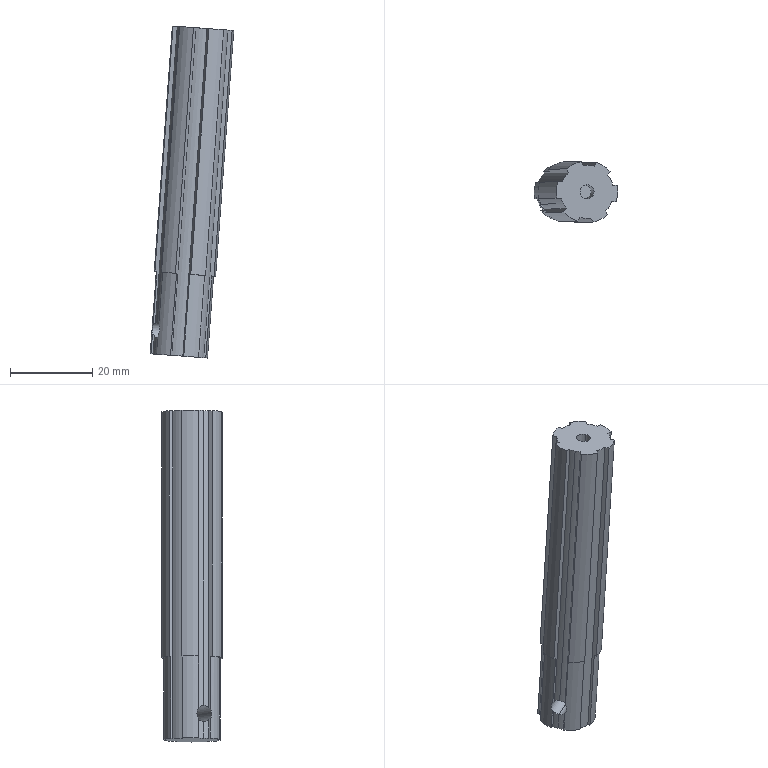Component | SolidWorks | DoubleFilmTransport-1_Spline-1 | 1 solid | 51 faces | volume 12069 mm3 | cylinder 26 | plane 25 | commonest cylinder face diameters 13 x10 15 x6 14 x6 3.4 x2 4 x2